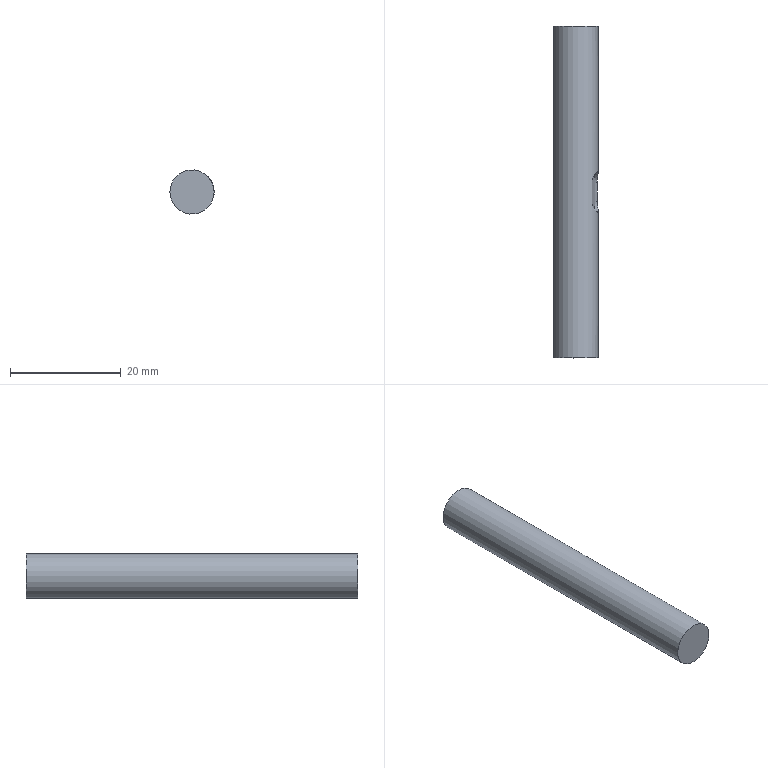Component | NX | 03E__27_2 | 1 solid | 8 faces | volume 2994 mm3 | plane 5 | cylinder 3 | commonest cylinder face diameters 3.996 x2 8 x1